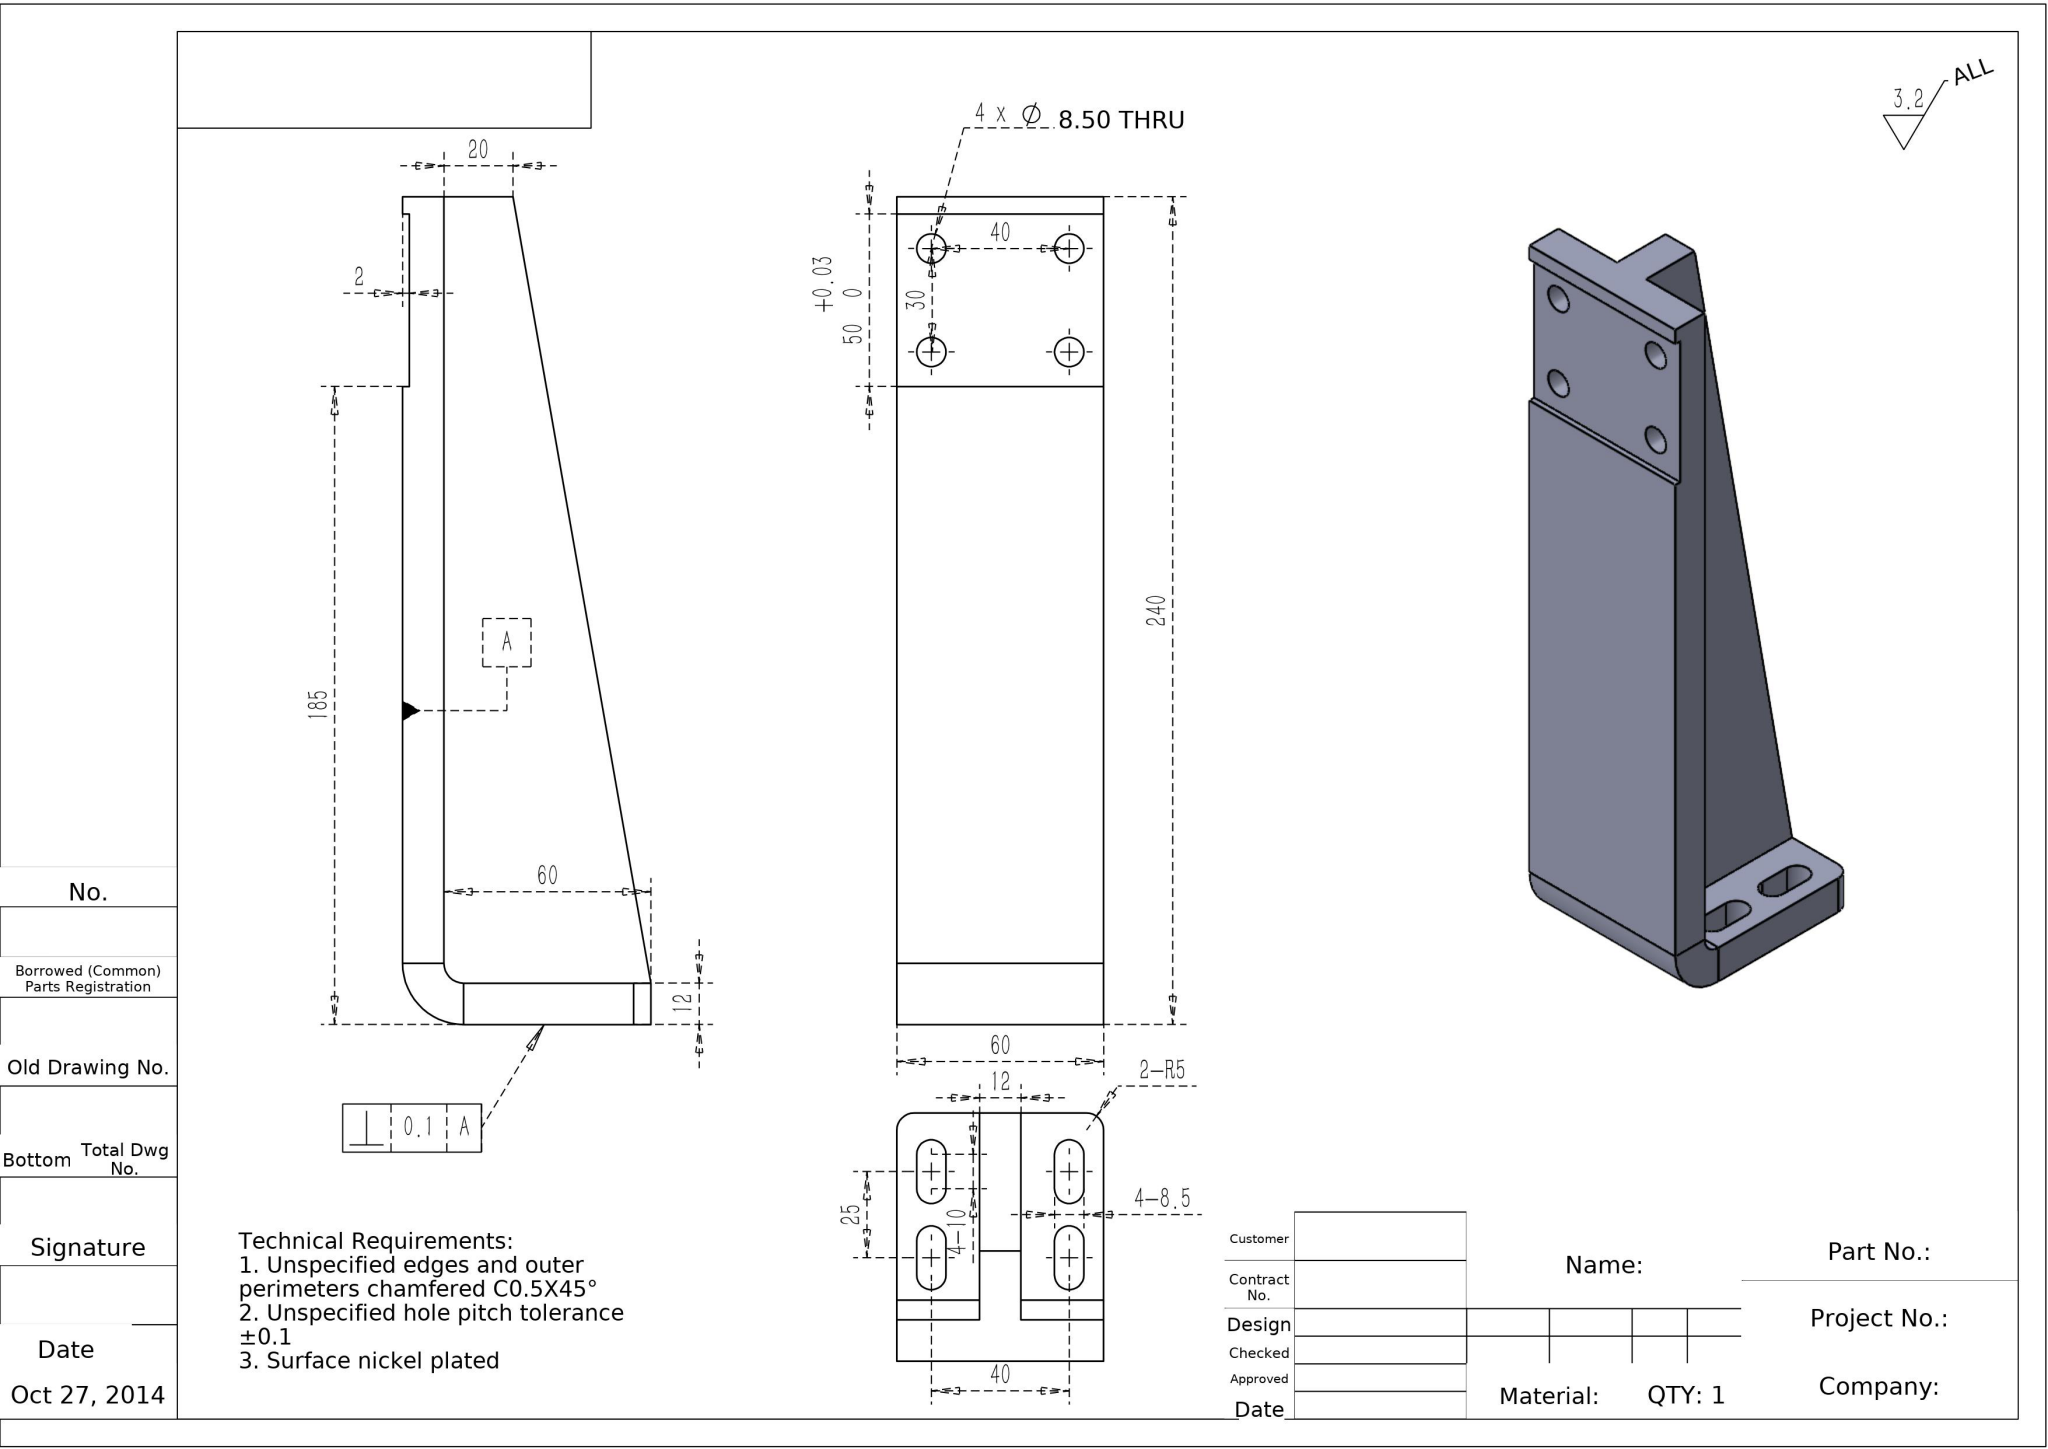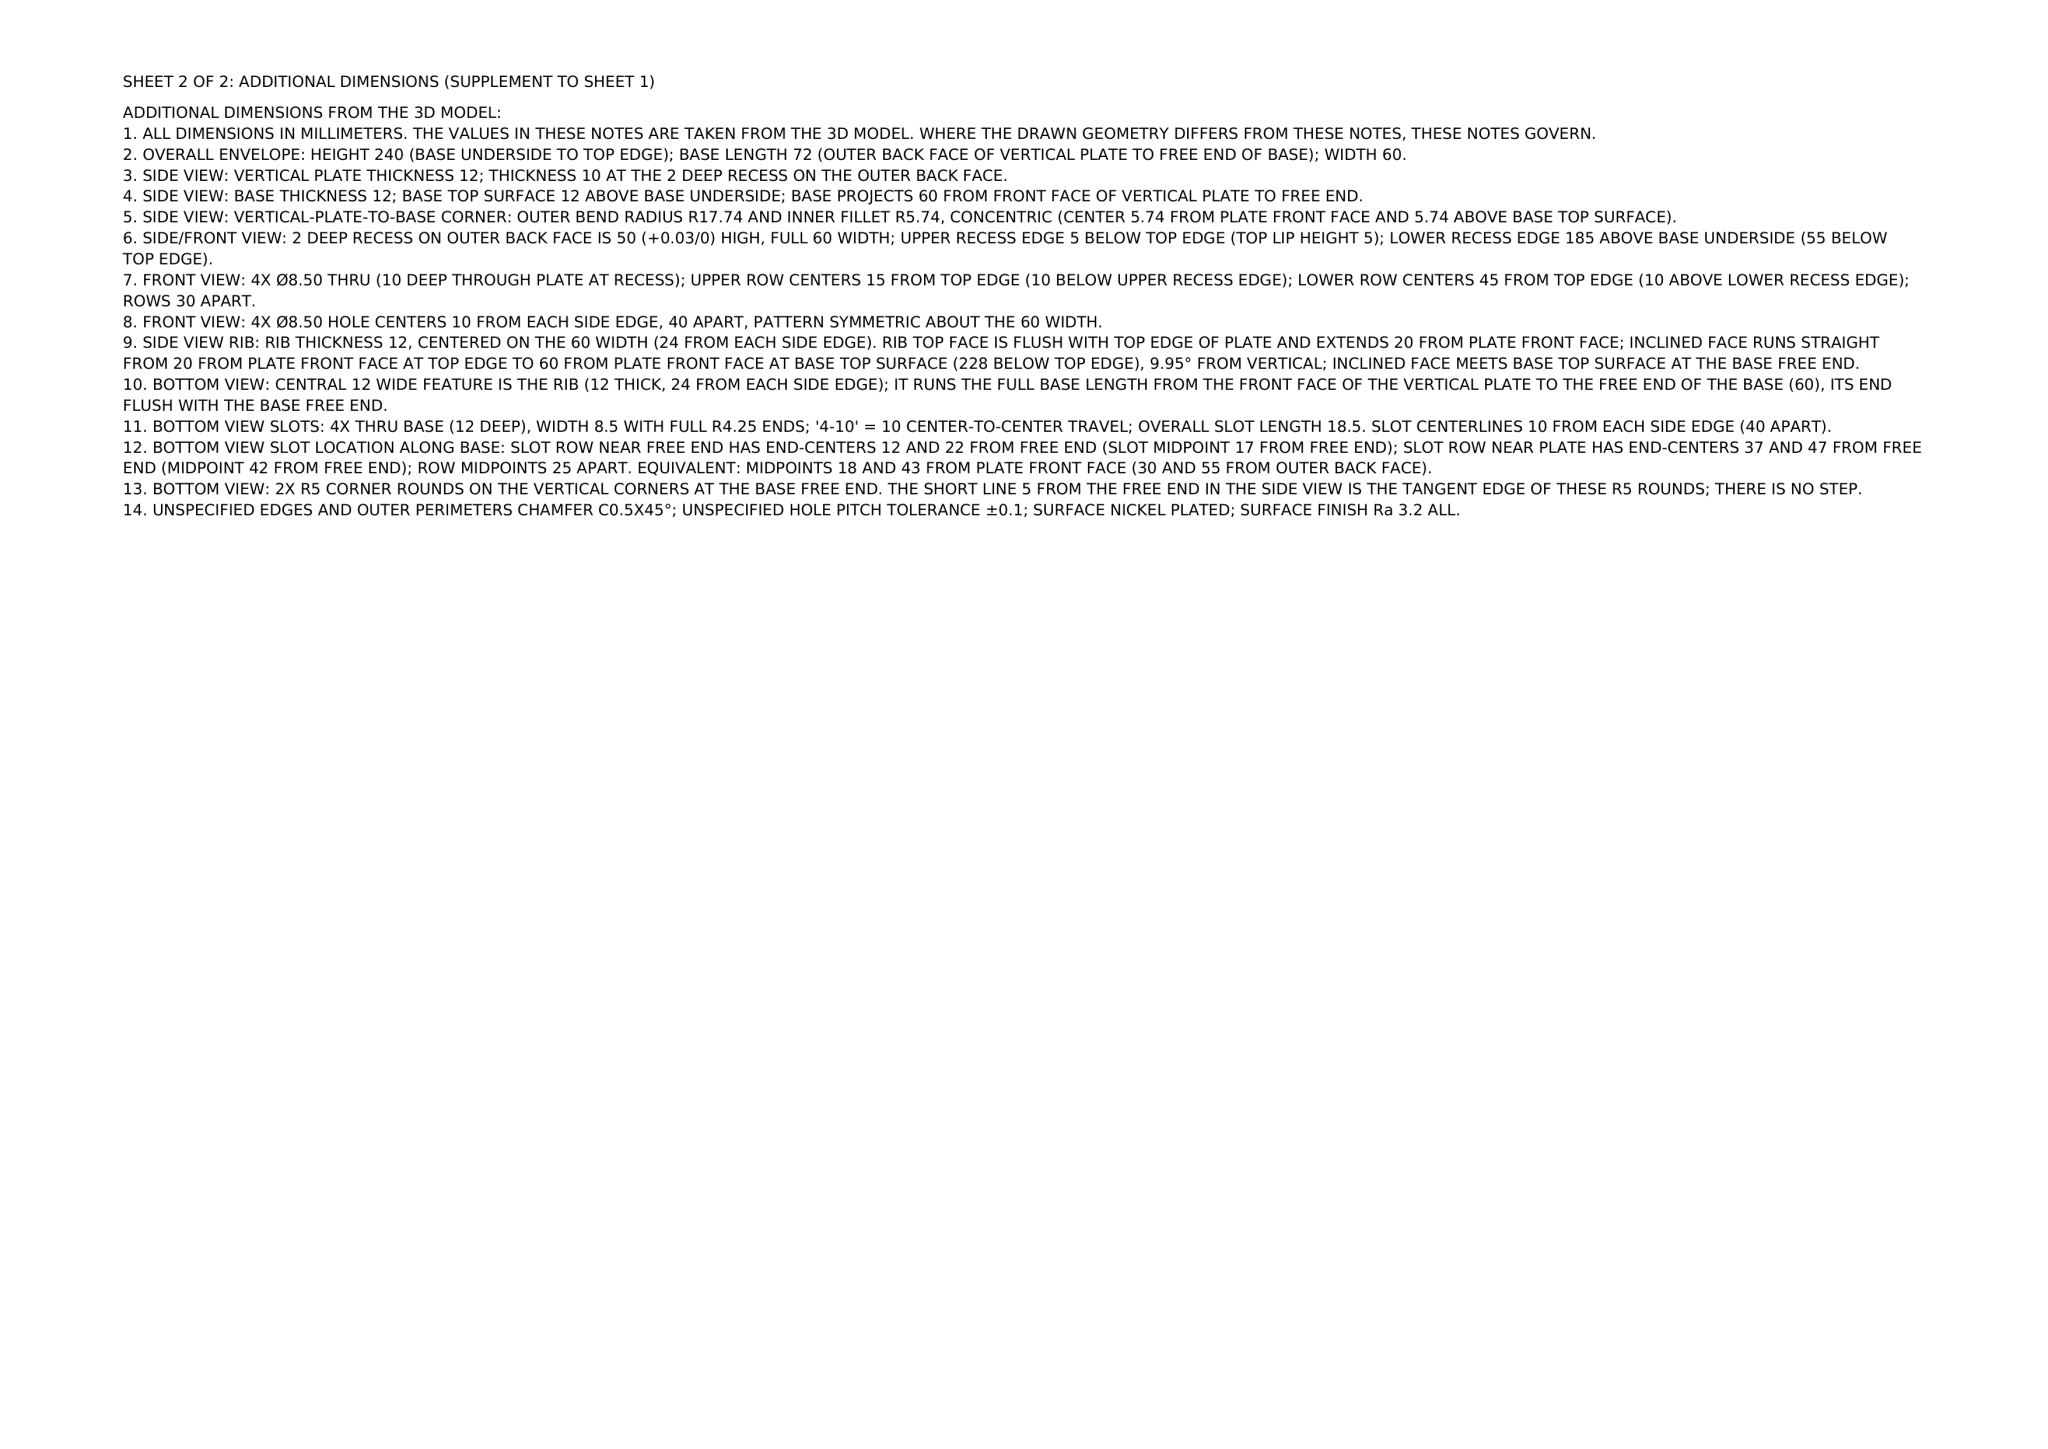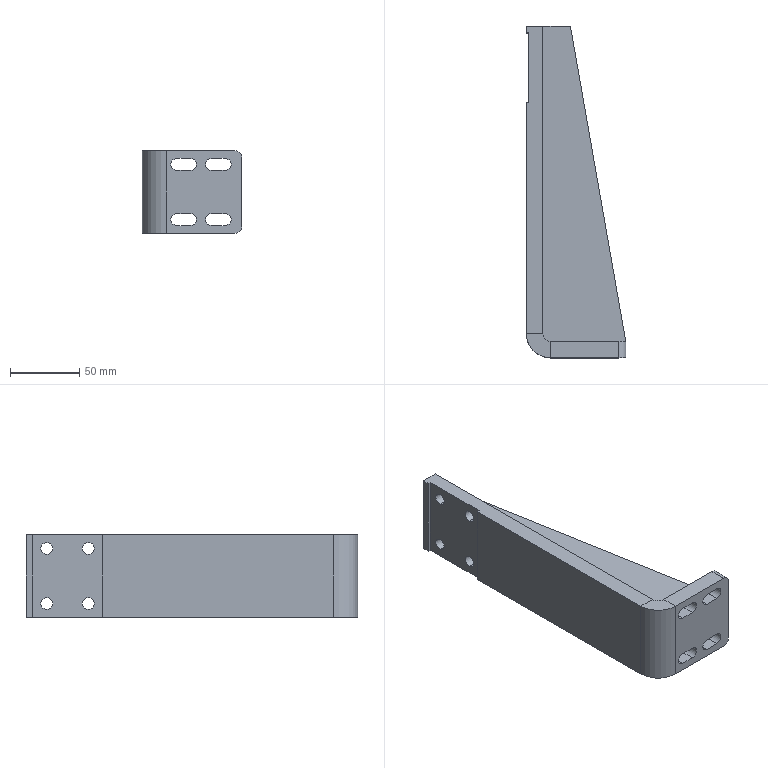Part | NX | mm | 1 solid | 50 faces | box 72 x 240 x 60 mm | volume 306526 mm3 | plane 29 | cylinder 21 | commonest cylinder face diameters 8.5 x16 11.473 x2 10 x2 35.473 x1